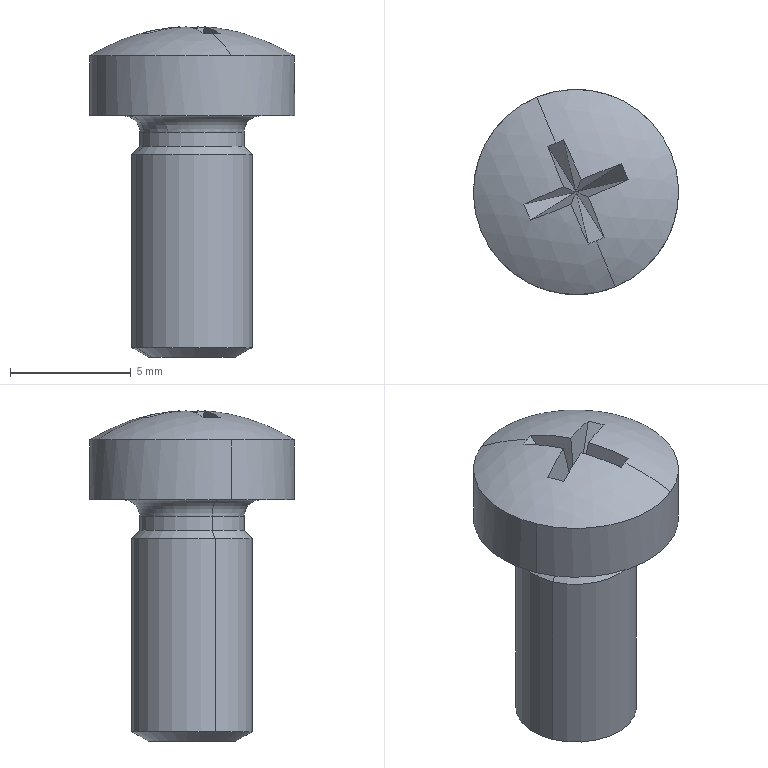Component | SolidWorks | GB_T818-2000PhillipsPanHeadScrewM5_10-2 | 1 solid | 28 faces | volume 359 mm3 | plane 14 | cylinder 6 | cone 4 | torus 2 | sphere 2 | commonest cylinder face diameters 4.33 x2 8.5 x2 5 x2